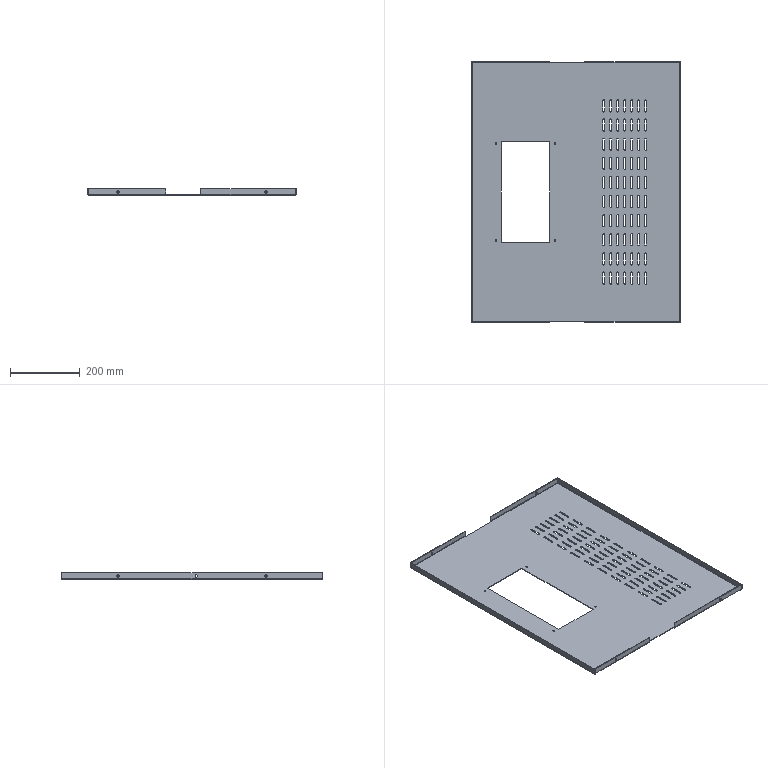Component | SolidWorks | BottomPlate(No.14)-1 | 1 solid | 440 faces | volume 867898 mm3 | cylinder 250 | plane 190 | commonest cylinder face diameters 5 x218 6.5 x20 6 x6 2 x6 | material Plain Carbon Steel